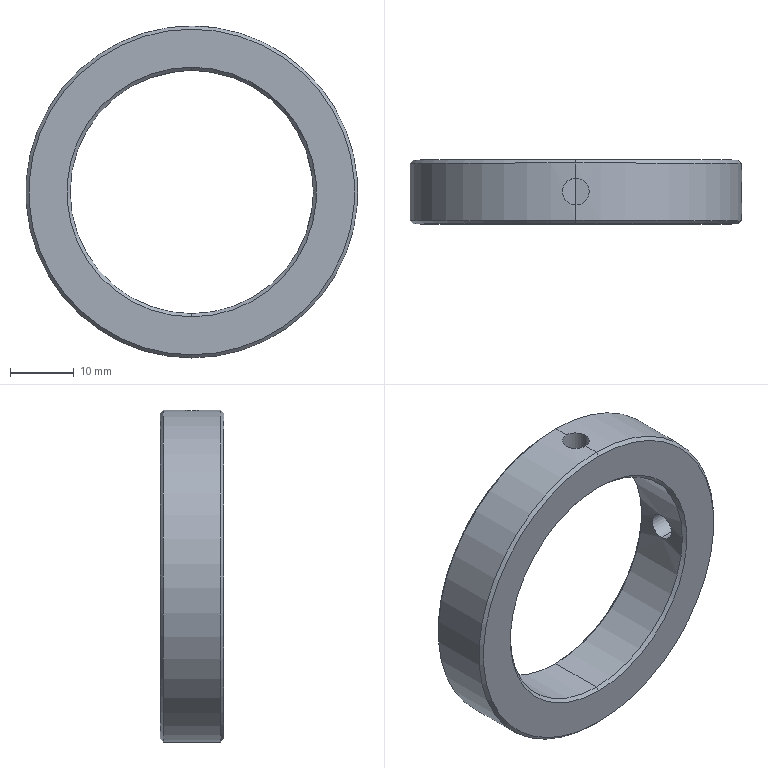Component | SolidWorks | 8TC-A15004-80-19A-1 | 1 solid | 18 faces | box 52 x 10 x 52 mm | volume 9573 mm3 | cylinder 8 | cone 8 | plane 2 | commonest cylinder face diameters 4.2 x4 38.1 x2 52 x2 | material Black Bakelite
build123d program:
from build123d import *

# Parameters (mm, degrees)
SKETCH1_R           = 26
SKETCH1_R_2         = 19.05
BOSS_EXTRUDE1_DEPTH = 5
CHAMFER1_SIZE       = 0.5
SKETCH2_W           = 2.1
SKETCH2_H           = 26
CIRPATTERN1_COUNT   = 2
CIRPATTERN1_ANGLE   = 90


with BuildPart() as part:
    # Sketch1 → Boss-Extrude1 (new, symmetric)
    with BuildSketch(Plane(origin=(0, 0, 0), x_dir=(1, 0, 0), z_dir=(0, 1, 0))):
        with Locations(Location((0, 0, 0), (0, 0, 270))):
            Circle(SKETCH1_R)
        with Locations(Location((0, 0, 0), (0, 0, 270))):
            Circle(SKETCH1_R_2, mode=Mode.SUBTRACT)
    extrude(amount=BOSS_EXTRUDE1_DEPTH, both=True)

    # Chamfer1
    chamfer1_edges = [part.edges().sort_by_distance(p)[0] for p in [
        (0, -5, -26),
        (0, 5, -26),
        (0, -5, -19.05),
        (0, 5, -19.05),
    ]]
    chamfer(chamfer1_edges, length=CHAMFER1_SIZE)

    # Sketch2 → M5 Tapped Hole1 (revolve, cut)
    with BuildSketch(Plane.ZX):
        with Locations((1.05, 13)):
            Rectangle(SKETCH2_W, SKETCH2_H)
    m5_tapped_hole1 = revolve(axis=Axis((-6.35, 0, 0), (1, 0, 0)), mode=Mode.SUBTRACT)

    # CirPattern1: M5 Tapped Hole1 ×2 about axis
    cirpattern1_axis = Axis((0, 5, 0), (0, -1, 0))
    for i in range(1, CIRPATTERN1_COUNT):
        add(m5_tapped_hole1.rotate(cirpattern1_axis, i * CIRPATTERN1_ANGLE / (CIRPATTERN1_COUNT - 1)), mode=Mode.SUBTRACT)


solid = part.part

# Placed as in the assembly
solid = solid.moved(Location((50, 188.5, -500), (0, 0, 0)))
STEP:
#1=CARTESIAN_POINT('',(2.051,7.421,-18.665));
#2=VERTEX_POINT('',#1);
#3=CARTESIAN_POINT('',(1.969,7.339,-18.661));
#4=VERTEX_POINT('',#3);
#5=CARTESIAN_POINT('',(2.051,7.421,-18.665));
#6=CARTESIAN_POINT('',(2.051,7.416,-18.665));
#7=CARTESIAN_POINT('',(2.051,7.41,-18.665));
#8=CARTESIAN_POINT('',(2.049,7.4,-18.665));
#9=CARTESIAN_POINT('',(2.047,7.395,-18.664));
#10=CARTESIAN_POINT('',(2.043,7.385,-18.664));
#11=CARTESIAN_POINT('',(2.04,7.38,-18.664));
#12=CARTESIAN_POINT('',(2.034,7.371,-18.664));
#13=CARTESIAN_POINT('',(2.031,7.367,-18.663));
#14=CARTESIAN_POINT('',(2.023,7.359,-18.663));
#15=CARTESIAN_POINT('',(2.019,7.356,-18.663));
#16=CARTESIAN_POINT('',(2.01,7.35,-18.662));
#17=CARTESIAN_POINT('',(2.005,7.347,-18.662));
#18=CARTESIAN_POINT('',(1.99,7.341,-18.662));
#19=CARTESIAN_POINT('',(1.979,7.339,-18.661));
#20=CARTESIAN_POINT('',(1.969,7.339,-18.661));
#21=B_SPLINE_CURVE_WITH_KNOTS('',3,(#5,#6,#7,#8,#9,#10,#11,#12,#13,#14,#15,#16,#17,#18,#19,#20),.UNSPECIFIED.,.F.,.F.,(4,2,2,2,2,2,2,4),(0.009853,0.01026,0.01067,0.01108,0.01149,0.0119,0.01231,0.01313),.UNSPECIFIED.);
#22=EDGE_CURVE('',#2,#4,#21,.T.);
#23=ORIENTED_EDGE('',*,*,#22,.F.);
#24=CARTESIAN_POINT('',(2.051,7.421,-18.94));
#25=VERTEX_POINT('',#24);
#26=CARTESIAN_POINT('',(2.051,7.421,-19.685));
#27=DIRECTION('',(0.,0.,-1.));
#28=VECTOR('',#27,39.37);
#29=LINE('',#26,#28);
#30=EDGE_CURVE('',#2,#25,#29,.T.);
#31=ORIENTED_EDGE('',*,*,#30,.T.);
#32=CARTESIAN_POINT('',(1.969,7.339,-18.935));
#33=VERTEX_POINT('',#32);
#34=CARTESIAN_POINT('',(2.051,7.421,-18.94));
#35=CARTESIAN_POINT('',(2.051,7.41,-18.94));
#36=CARTESIAN_POINT('',(2.049,7.4,-18.939));
#37=CARTESIAN_POINT('',(2.041,7.38,-18.939));
#38=CARTESIAN_POINT('',(2.035,7.37,-18.938));
#39=CARTESIAN_POINT('',(2.023,7.359,-18.937));
#40=CARTESIAN_POINT('',(2.019,7.356,-18.937));
#41=CARTESIAN_POINT('',(2.01,7.35,-18.936));
#42=CARTESIAN_POINT('',(2.005,7.347,-18.936));
#43=CARTESIAN_POINT('',(1.995,7.343,-18.935));
#44=CARTESIAN_POINT('',(1.99,7.341,-18.935));
#45=CARTESIAN_POINT('',(1.979,7.339,-18.935));
#46=CARTESIAN_POINT('',(1.974,7.339,-18.935));
#47=CARTESIAN_POINT('',(1.969,7.339,-18.935));
#48=B_SPLINE_CURVE_WITH_KNOTS('',3,(#34,#35,#36,#37,#38,#39,#40,#41,#42,#43,#44,#45,#46,#47),.UNSPECIFIED.,.F.,.F.,(4,2,2,2,2,2,4),(0.006571,0.007392,0.008214,0.008624,0.009035,0.009446,0.009857),.UNSPECIFIED.);
#49=EDGE_CURVE('',#25,#33,#48,.T.);
#50=ORIENTED_EDGE('',*,*,#49,.T.);
#51=CARTESIAN_POINT('',(1.886,7.421,-18.94));
#52=VERTEX_POINT('',#51);
#53=CARTESIAN_POINT('',(1.969,7.339,-18.935));
#54=CARTESIAN_POINT('',(1.963,7.339,-18.935));
#55=CARTESIAN_POINT('',(1.958,7.339,-18.935));
#56=CARTESIAN_POINT('',(1.947,7.341,-18.935));
#57=CARTESIAN_POINT('',(1.942,7.343,-18.935));
#58=CARTESIAN_POINT('',(1.932,7.347,-18.936));
#59=CARTESIAN_POINT('',(1.927,7.349,-18.936));
#60=CARTESIAN_POINT('',(1.918,7.355,-18.937));
#61=CARTESIAN_POINT('',(1.914,7.359,-18.937));
#62=CARTESIAN_POINT('',(1.902,7.37,-18.938));
#63=CARTESIAN_POINT('',(1.896,7.38,-18.939));
#64=CARTESIAN_POINT('',(1.888,7.399,-18.939));
#65=CARTESIAN_POINT('',(1.886,7.41,-18.94));
#66=CARTESIAN_POINT('',(1.886,7.421,-18.94));
#67=B_SPLINE_CURVE_WITH_KNOTS('',3,(#53,#54,#55,#56,#57,#58,#59,#60,#61,#62,#63,#64,#65,#66),.UNSPECIFIED.,.F.,.F.,(4,2,2,2,2,2,4),(0.009857,0.01027,0.01068,0.01109,0.0115,0.01232,0.01314),.UNSPECIFIED.);
#68=EDGE_CURVE('',#33,#52,#67,.T.);
#69=ORIENTED_EDGE('',*,*,#68,.T.);
#70=CARTESIAN_POINT('',(1.886,7.421,-18.665));
#71=VERTEX_POINT('',#70);
#72=CARTESIAN_POINT('',(1.886,7.421,-19.685));
#73=DIRECTION('',(0.,0.,-1.));
#74=VECTOR('',#73,39.37);
#75=LINE('',#72,#74);
#76=EDGE_CURVE('',#71,#52,#75,.T.);
#77=ORIENTED_EDGE('',*,*,#76,.F.);
#78=CARTESIAN_POINT('',(1.969,7.339,-18.661));
#79=CARTESIAN_POINT('',(1.963,7.339,-18.661));
#80=CARTESIAN_POINT('',(1.958,7.339,-18.661));
#81=CARTESIAN_POINT('',(1.947,7.341,-18.662));
#82=CARTESIAN_POINT('',(1.942,7.343,-18.662));
#83=CARTESIAN_POINT('',(1.932,7.347,-18.662));
#84=CARTESIAN_POINT('',(1.927,7.35,-18.662));
#85=CARTESIAN_POINT('',(1.918,7.356,-18.663));
#86=CARTESIAN_POINT('',(1.914,7.359,-18.663));
#87=CARTESIAN_POINT('',(1.902,7.37,-18.664));
#88=CARTESIAN_POINT('',(1.896,7.38,-18.664));
#89=CARTESIAN_POINT('',(1.888,7.4,-18.665));
#90=CARTESIAN_POINT('',(1.886,7.41,-18.665));
#91=CARTESIAN_POINT('',(1.886,7.421,-18.665));
#92=B_SPLINE_CURVE_WITH_KNOTS('',3,(#78,#79,#80,#81,#82,#83,#84,#85,#86,#87,#88,#89,#90,#91),.UNSPECIFIED.,.F.,.F.,(4,2,2,2,2,2,4),(0.,0.0004106,0.0008212,0.001232,0.001642,0.002464,0.003285),.UNSPECIFIED.);
#93=EDGE_CURVE('',#4,#71,#92,.T.);
#94=ORIENTED_EDGE('',*,*,#93,.F.);
#95=EDGE_LOOP('',(#23,#31,#50,#69,#77,#94));
#96=FACE_OUTER_BOUND('',#95,.T.);
#97=CARTESIAN_POINT('',(1.969,7.421,-19.685));
#98=DIRECTION('',(0.,0.,-1.));
#99=DIRECTION('',(-1.,0.,0.));
#100=AXIS2_PLACEMENT_3D('',#97,#98,#99);
#101=CYLINDRICAL_SURFACE('',#100,0.08268);
#102=ADVANCED_FACE('',(#96),#101,.F.);
#103=CARTESIAN_POINT('',(2.989,7.421,-19.768));
#104=VERTEX_POINT('',#103);
#105=CARTESIAN_POINT('',(2.989,7.421,-19.602));
#106=VERTEX_POINT('',#105);
#107=CARTESIAN_POINT('',(2.989,7.421,-19.768));
#108=CARTESIAN_POINT('',(2.989,7.416,-19.768));
#109=CARTESIAN_POINT('',(2.989,7.41,-19.767));
#110=CARTESIAN_POINT('',(2.989,7.4,-19.765));
#111=CARTESIAN_POINT('',(2.989,7.395,-19.763));
#112=CARTESIAN_POINT('',(2.989,7.385,-19.759));
#113=CARTESIAN_POINT('',(2.99,7.38,-19.757));
#114=CARTESIAN_POINT('',(2.99,7.371,-19.751));
#115=CARTESIAN_POINT('',(2.99,7.367,-19.747));
#116=CARTESIAN_POINT('',(2.991,7.359,-19.74));
#117=CARTESIAN_POINT('',(2.991,7.356,-19.736));
#118=CARTESIAN_POINT('',(2.991,7.35,-19.726));
#119=CARTESIAN_POINT('',(2.991,7.347,-19.722));
#120=CARTESIAN_POINT('',(2.992,7.341,-19.707));
#121=CARTESIAN_POINT('',(2.992,7.339,-19.696));
#122=CARTESIAN_POINT('',(2.992,7.339,-19.68));
#123=CARTESIAN_POINT('',(2.992,7.339,-19.674));
#124=CARTESIAN_POINT('',(2.992,7.341,-19.664));
#125=CARTESIAN_POINT('',(2.992,7.343,-19.658));
#126=CARTESIAN_POINT('',(2.991,7.347,-19.648));
#127=CARTESIAN_POINT('',(2.991,7.35,-19.644));
#128=CARTESIAN_POINT('',(2.991,7.356,-19.635));
#129=CARTESIAN_POINT('',(2.991,7.359,-19.63));
#130=CARTESIAN_POINT('',(2.99,7.37,-19.619));
#131=CARTESIAN_POINT('',(2.99,7.38,-19.613));
#132=CARTESIAN_POINT('',(2.989,7.4,-19.605));
#133=CARTESIAN_POINT('',(2.989,7.41,-19.602));
#134=CARTESIAN_POINT('',(2.989,7.421,-19.602));
#135=B_SPLINE_CURVE_WITH_KNOTS('',3,(#107,#108,#109,#110,#111,#112,#113,#114,#115,#116,#117,#118,#119,#120,#121,#122,#123,#124,#125,#126,#127,#128,#129,#130,#131,#132,#133,#134),.UNSPECIFIED.,.F.,.F.,(4,2,2,2,2,2,2,2,2,2,2,2,2,4),(0.009853,0.01026,0.01067,0.01108,0.01149,0.01191,0.01232,0.01314,0.01355,0.01396,0.01437,0.01478,0.0156,0.01642),.UNSPECIFIED.);
#136=EDGE_CURVE('',#104,#106,#135,.T.);
#137=ORIENTED_EDGE('',*,*,#136,.F.);
#138=CARTESIAN_POINT('',(2.714,7.421,-19.768));
#139=VERTEX_POINT('',#138);
#140=CARTESIAN_POINT('',(1.969,7.421,-19.768));
#141=DIRECTION('',(-1.,0.,0.));
#142=VECTOR('',#141,39.37);
#143=LINE('',#140,#142);
#144=EDGE_CURVE('',#104,#139,#143,.T.);
#145=ORIENTED_EDGE('',*,*,#144,.T.);
#146=CARTESIAN_POINT('',(2.714,7.421,-19.602));
#147=VERTEX_POINT('',#146);
#148=CARTESIAN_POINT('',(2.714,7.421,-19.768));
#149=CARTESIAN_POINT('',(2.714,7.41,-19.768));
#150=CARTESIAN_POINT('',(2.714,7.4,-19.766));
#151=CARTESIAN_POINT('',(2.715,7.38,-19.757));
#152=CARTESIAN_POINT('',(2.716,7.37,-19.751));
#153=CARTESIAN_POINT('',(2.717,7.359,-19.74));
#154=CARTESIAN_POINT('',(2.717,7.356,-19.735));
#155=CARTESIAN_POINT('',(2.717,7.35,-19.727));
#156=CARTESIAN_POINT('',(2.718,7.347,-19.722));
#157=CARTESIAN_POINT('',(2.718,7.343,-19.712));
#158=CARTESIAN_POINT('',(2.718,7.341,-19.707));
#159=CARTESIAN_POINT('',(2.718,7.339,-19.696));
#160=CARTESIAN_POINT('',(2.719,7.339,-19.691));
#161=CARTESIAN_POINT('',(2.719,7.339,-19.68));
#162=CARTESIAN_POINT('',(2.718,7.339,-19.674));
#163=CARTESIAN_POINT('',(2.718,7.341,-19.664));
#164=CARTESIAN_POINT('',(2.718,7.343,-19.658));
#165=CARTESIAN_POINT('',(2.718,7.347,-19.648));
#166=CARTESIAN_POINT('',(2.717,7.349,-19.644));
#167=CARTESIAN_POINT('',(2.717,7.355,-19.635));
#168=CARTESIAN_POINT('',(2.717,7.359,-19.63));
#169=CARTESIAN_POINT('',(2.716,7.37,-19.619));
#170=CARTESIAN_POINT('',(2.715,7.38,-19.613));
#171=CARTESIAN_POINT('',(2.714,7.399,-19.605));
#172=CARTESIAN_POINT('',(2.714,7.41,-19.602));
#173=CARTESIAN_POINT('',(2.714,7.421,-19.602));
#174=B_SPLINE_CURVE_WITH_KNOTS('',3,(#148,#149,#150,#151,#152,#153,#154,#155,#156,#157,#158,#159,#160,#161,#162,#163,#164,#165,#166,#167,#168,#169,#170,#171,#172,#173),.UNSPECIFIED.,.F.,.F.,(4,2,2,2,2,2,2,2,2,2,2,2,4),(0.006571,0.007392,0.008213,0.008623,0.009034,0.009444,0.009855,0.01027,0.01068,0.01109,0.0115,0.01232,0.01314),.UNSPECIFIED.);
#175=EDGE_CURVE('',#139,#147,#174,.T.);
#176=ORIENTED_EDGE('',*,*,#175,.T.);
#177=CARTESIAN_POINT('',(1.969,7.421,-19.602));
#178=DIRECTION('',(-1.,0.,0.));
#179=VECTOR('',#178,39.37);
#180=LINE('',#177,#179);
#181=EDGE_CURVE('',#106,#147,#180,.T.);
#182=ORIENTED_EDGE('',*,*,#181,.F.);
#183=EDGE_LOOP('',(#137,#145,#176,#182));
#184=FACE_OUTER_BOUND('',#183,.T.);
#185=CARTESIAN_POINT('',(1.969,7.421,-19.685));
#186=DIRECTION('',(-1.,0.,0.));
#187=DIRECTION('',(0.,0.,1.));
#188=AXIS2_PLACEMENT_3D('',#185,#186,#187);
#189=CYLINDRICAL_SURFACE('',#188,0.08268);
#190=ADVANCED_FACE('',(#184),#189,.F.);
#191=CARTESIAN_POINT('',(1.969,7.244,-18.935));
#192=VERTEX_POINT('',#191);
#193=CARTESIAN_POINT('',(1.969,7.244,-20.435));
#194=VERTEX_POINT('',#193);
#195=CARTESIAN_POINT('',(1.969,7.244,-19.685));
#196=DIRECTION('',(0.,-1.,0.));
#197=DIRECTION('',(0.,0.,1.));
#198=AXIS2_PLACEMENT_3D('',#195,#196,#197);
#199=CIRCLE('',#198,0.75);
#200=EDGE_CURVE('',#192,#194,#199,.T.);
#201=ORIENTED_EDGE('',*,*,#200,.F.);
#202=CARTESIAN_POINT('',(1.969,7.224,-18.915));
#203=VERTEX_POINT('',#202);
#204=CARTESIAN_POINT('',(1.969,7.224,-18.915));
#205=DIRECTION('',(0.,-0.7071,0.7071));
#206=VECTOR('',#205,39.37);
#207=LINE('',#204,#206);
#208=EDGE_CURVE('',#192,#203,#207,.T.);
#209=ORIENTED_EDGE('',*,*,#208,.T.);
#210=CARTESIAN_POINT('',(1.969,7.224,-20.455));
#211=VERTEX_POINT('',#210);
#212=CARTESIAN_POINT('',(1.969,7.224,-19.685));
#213=DIRECTION('',(0.,1.,0.));
#214=DIRECTION('',(0.,0.,1.));
#215=AXIS2_PLACEMENT_3D('',#212,#213,#214);
#216=CIRCLE('',#215,0.7697);
#217=EDGE_CURVE('',#211,#203,#216,.T.);
#218=ORIENTED_EDGE('',*,*,#217,.F.);
#219=CARTESIAN_POINT('',(1.969,7.224,-20.455));
#220=DIRECTION('',(0.,-0.7071,-0.7071));
#221=VECTOR('',#220,39.37);
#222=LINE('',#219,#221);
#223=EDGE_CURVE('',#194,#211,#222,.T.);
#224=ORIENTED_EDGE('',*,*,#223,.F.);
#225=EDGE_LOOP('',(#201,#209,#218,#224));
#226=FACE_OUTER_BOUND('',#225,.T.);
#227=CARTESIAN_POINT('',(1.969,7.224,-19.685));
#228=DIRECTION('',(0.,-1.,0.));
#229=DIRECTION('',(0.,0.,-1.));
#230=AXIS2_PLACEMENT_3D('',#227,#228,#229);
#231=CONICAL_SURFACE('',#230,0.7697,0.7854);
#232=ADVANCED_FACE('',(#226),#231,.F.);
#233=CARTESIAN_POINT('',(1.969,7.224,-20.689));
#234=VERTEX_POINT('',#233);
#235=CARTESIAN_POINT('',(1.969,7.224,-18.681));
#236=VERTEX_POINT('',#235);
#237=CARTESIAN_POINT('',(1.969,7.224,-19.685));
#238=DIRECTION('',(0.,-1.,0.));
#239=DIRECTION('',(0.,0.,1.));
#240=AXIS2_PLACEMENT_3D('',#237,#238,#239);
#241=CIRCLE('',#240,1.004);
#242=EDGE_CURVE('',#234,#236,#241,.T.);
#243=ORIENTED_EDGE('',*,*,#242,.F.);
#244=CARTESIAN_POINT('',(1.969,7.244,-20.709));
#245=VERTEX_POINT('',#244);
#246=CARTESIAN_POINT('',(1.969,7.244,-20.709));
#247=DIRECTION('',(0.,0.7071,-0.7071));
#248=VECTOR('',#247,39.37);
#249=LINE('',#246,#248);
#250=EDGE_CURVE('',#234,#245,#249,.T.);
#251=ORIENTED_EDGE('',*,*,#250,.T.);
#252=CARTESIAN_POINT('',(1.969,7.244,-18.661));
#253=VERTEX_POINT('',#252);
#254=CARTESIAN_POINT('',(1.969,7.244,-19.685));
#255=DIRECTION('',(0.,1.,0.));
#256=DIRECTION('',(0.,0.,1.));
#257=AXIS2_PLACEMENT_3D('',#254,#255,#256);
#258=CIRCLE('',#257,1.024);
#259=EDGE_CURVE('',#253,#245,#258,.T.);
#260=ORIENTED_EDGE('',*,*,#259,.F.);
#261=CARTESIAN_POINT('',(1.969,7.244,-18.661));
#262=DIRECTION('',(0.,0.7071,0.7071));
#263=VECTOR('',#262,39.37);
#264=LINE('',#261,#263);
#265=EDGE_CURVE('',#236,#253,#264,.T.);
#266=ORIENTED_EDGE('',*,*,#265,.F.);
#267=EDGE_LOOP('',(#243,#251,#260,#266));
#268=FACE_OUTER_BOUND('',#267,.T.);
#269=CARTESIAN_POINT('',(1.969,7.244,-19.685));
#270=DIRECTION('',(0.,1.,0.));
#271=DIRECTION('',(0.,0.,1.));
#272=AXIS2_PLACEMENT_3D('',#269,#270,#271);
#273=CONICAL_SURFACE('',#272,1.024,0.7854);
#274=ADVANCED_FACE('',(#268),#273,.T.);
#275=CARTESIAN_POINT('',(1.969,7.618,-18.681));
#276=VERTEX_POINT('',#275);
#277=CARTESIAN_POINT('',(1.969,7.618,-20.689));
#278=VERTEX_POINT('',#277);
#279=CARTESIAN_POINT('',(1.969,7.618,-19.685));
#280=DIRECTION('',(0.,1.,0.));
#281=DIRECTION('',(0.,0.,1.));
#282=AXIS2_PLACEMENT_3D('',#279,#280,#281);
#283=CIRCLE('',#282,1.004);
#284=EDGE_CURVE('',#276,#278,#283,.T.);
#285=ORIENTED_EDGE('',*,*,#284,.F.);
#286=CARTESIAN_POINT('',(1.969,7.598,-18.661));
#287=VERTEX_POINT('',#286);
#288=CARTESIAN_POINT('',(1.969,7.618,-18.681));
#289=DIRECTION('',(0.,-0.7071,0.7071));
#290=VECTOR('',#289,39.37);
#291=LINE('',#288,#290);
#292=EDGE_CURVE('',#276,#287,#291,.T.);
#293=ORIENTED_EDGE('',*,*,#292,.T.);
#294=CARTESIAN_POINT('',(1.969,7.598,-20.709));
#295=VERTEX_POINT('',#294);
#296=CARTESIAN_POINT('',(1.969,7.598,-19.685));
#297=DIRECTION('',(0.,-1.,0.));
#298=DIRECTION('',(0.,0.,1.));
#299=AXIS2_PLACEMENT_3D('',#296,#297,#298);
#300=CIRCLE('',#299,1.024);
#301=EDGE_CURVE('',#295,#287,#300,.T.);
#302=ORIENTED_EDGE('',*,*,#301,.F.);
#303=CARTESIAN_POINT('',(1.969,7.618,-20.689));
#304=DIRECTION('',(0.,-0.7071,-0.7071));
#305=VECTOR('',#304,39.37);
#306=LINE('',#303,#305);
#307=EDGE_CURVE('',#278,#295,#306,.T.);
#308=ORIENTED_EDGE('',*,*,#307,.F.);
#309=EDGE_LOOP('',(#285,#293,#302,#308));
#310=FACE_OUTER_BOUND('',#309,.T.);
#311=CARTESIAN_POINT('',(1.969,7.618,-19.685));
#312=DIRECTION('',(0.,-1.,0.));
#313=DIRECTION('',(0.,0.,-1.));
#314=AXIS2_PLACEMENT_3D('',#311,#312,#313);
#315=CONICAL_SURFACE('',#314,1.004,0.7854);
#316=ADVANCED_FACE('',(#310),#315,.T.);
#317=CARTESIAN_POINT('',(1.969,7.598,-20.435));
#318=VERTEX_POINT('',#317);
#319=CARTESIAN_POINT('',(1.969,7.598,-18.935));
#320=VERTEX_POINT('',#319);
#321=CARTESIAN_POINT('',(1.969,7.598,-19.685));
#322=DIRECTION('',(0.,1.,0.));
#323=DIRECTION('',(0.,0.,1.));
#324=AXIS2_PLACEMENT_3D('',#321,#322,#323);
#325=CIRCLE('',#324,0.75);
#326=EDGE_CURVE('',#318,#320,#325,.T.);
#327=ORIENTED_EDGE('',*,*,#326,.F.);
#328=CARTESIAN_POINT('',(1.969,7.618,-20.455));
#329=VERTEX_POINT('',#328);
#330=CARTESIAN_POINT('',(1.969,7.598,-20.435));
#331=DIRECTION('',(0.,0.7071,-0.7071));
#332=VECTOR('',#331,39.37);
#333=LINE('',#330,#332);
#334=EDGE_CURVE('',#318,#329,#333,.T.);
#335=ORIENTED_EDGE('',*,*,#334,.T.);
#336=CARTESIAN_POINT('',(1.969,7.618,-18.915));
#337=VERTEX_POINT('',#336);
#338=CARTESIAN_POINT('',(1.969,7.618,-19.685));
#339=DIRECTION('',(0.,-1.,0.));
#340=DIRECTION('',(0.,0.,1.));
#341=AXIS2_PLACEMENT_3D('',#338,#339,#340);
#342=CIRCLE('',#341,0.7697);
#343=EDGE_CURVE('',#337,#329,#342,.T.);
#344=ORIENTED_EDGE('',*,*,#343,.F.);
#345=CARTESIAN_POINT('',(1.969,7.598,-18.935));
#346=DIRECTION('',(0.,0.7071,0.7071));
#347=VECTOR('',#346,39.37);
#348=LINE('',#345,#347);
#349=EDGE_CURVE('',#320,#337,#348,.T.);
#350=ORIENTED_EDGE('',*,*,#349,.F.);
#351=EDGE_LOOP('',(#327,#335,#344,#350));
#352=FACE_OUTER_BOUND('',#351,.T.);
#353=CARTESIAN_POINT('',(1.969,7.598,-19.685));
#354=DIRECTION('',(0.,1.,0.));
#355=DIRECTION('',(0.,0.,1.));
#356=AXIS2_PLACEMENT_3D('',#353,#354,#355);
#357=CONICAL_SURFACE('',#356,0.75,0.7854);
#358=ADVANCED_FACE('',(#352),#357,.F.);
#359=ORIENTED_EDGE('',*,*,#326,.T.);
#360=CARTESIAN_POINT('',(1.969,7.504,-18.935));
#361=VERTEX_POINT('',#360);
#362=CARTESIAN_POINT('',(1.969,7.618,-18.935));
#363=DIRECTION('',(0.,-1.,0.));
#364=VECTOR('',#363,39.37);
#365=LINE('',#362,#364);
#366=EDGE_CURVE('',#320,#361,#365,.T.);
#367=ORIENTED_EDGE('',*,*,#366,.T.);
#368=CARTESIAN_POINT('',(1.886,7.421,-18.94));
#369=CARTESIAN_POINT('',(1.886,7.427,-18.94));
#370=CARTESIAN_POINT('',(1.886,7.432,-18.94));
#371=CARTESIAN_POINT('',(1.888,7.443,-18.939));
#372=CARTESIAN_POINT('',(1.89,7.448,-18.939));
#373=CARTESIAN_POINT('',(1.894,7.458,-18.939));
#374=CARTESIAN_POINT('',(1.897,7.463,-18.938));
#375=CARTESIAN_POINT('',(1.903,7.472,-18.938));
#376=CARTESIAN_POINT('',(1.906,7.476,-18.938));
#377=CARTESIAN_POINT('',(1.918,7.487,-18.937));
#378=CARTESIAN_POINT('',(1.927,7.494,-18.936));
#379=CARTESIAN_POINT('',(1.947,7.502,-18.935));
#380=CARTESIAN_POINT('',(1.958,7.504,-18.935));
#381=CARTESIAN_POINT('',(1.969,7.504,-18.935));
#382=B_SPLINE_CURVE_WITH_KNOTS('',3,(#368,#369,#370,#371,#372,#373,#374,#375,#376,#377,#378,#379,#380,#381),.UNSPECIFIED.,.F.,.F.,(4,2,2,2,2,2,4),(0.,0.0004108,0.0008215,0.001232,0.001643,0.002465,0.003286),.UNSPECIFIED.);
#383=EDGE_CURVE('',#52,#361,#382,.T.);
#384=ORIENTED_EDGE('',*,*,#383,.F.);
#385=ORIENTED_EDGE('',*,*,#68,.F.);
#386=CARTESIAN_POINT('',(1.969,7.618,-18.935));
#387=DIRECTION('',(0.,-1.,0.));
#388=VECTOR('',#387,39.37);
#389=LINE('',#386,#388);
#390=EDGE_CURVE('',#33,#192,#389,.T.);
#391=ORIENTED_EDGE('',*,*,#390,.T.);
#392=ORIENTED_EDGE('',*,*,#200,.T.);
#393=CARTESIAN_POINT('',(1.969,7.618,-20.435));
#394=DIRECTION('',(0.,-1.,0.));
#395=VECTOR('',#394,39.37);
#396=LINE('',#393,#395);
#397=EDGE_CURVE('',#318,#194,#396,.T.);
#398=ORIENTED_EDGE('',*,*,#397,.F.);
#399=EDGE_LOOP('',(#359,#367,#384,#385,#391,#392,#398));
#400=FACE_OUTER_BOUND('',#399,.T.);
#401=CARTESIAN_POINT('',(1.969,7.618,-19.685));
#402=DIRECTION('',(0.,-1.,0.));
#403=DIRECTION('',(0.,0.,-1.));
#404=AXIS2_PLACEMENT_3D('',#401,#402,#403);
#405=CYLINDRICAL_SURFACE('',#404,0.75);
#406=ADVANCED_FACE('',(#400),#405,.F.);
#407=CARTESIAN_POINT('',(2.989,7.421,-19.602));
#408=CARTESIAN_POINT('',(2.989,7.427,-19.602));
#409=CARTESIAN_POINT('',(2.989,7.432,-19.603));
#410=CARTESIAN_POINT('',(2.989,7.443,-19.605));
#411=CARTESIAN_POINT('',(2.989,7.448,-19.607));
#412=CARTESIAN_POINT('',(2.989,7.458,-19.611));
#413=CARTESIAN_POINT('',(2.99,7.463,-19.613));
#414=CARTESIAN_POINT('',(2.99,7.472,-19.619));
#415=CARTESIAN_POINT('',(2.99,7.476,-19.623));
#416=CARTESIAN_POINT('',(2.991,7.484,-19.63));
#417=CARTESIAN_POINT('',(2.991,7.487,-19.635));
#418=CARTESIAN_POINT('',(2.991,7.493,-19.644));
#419=CARTESIAN_POINT('',(2.991,7.496,-19.648));
#420=CARTESIAN_POINT('',(2.992,7.5,-19.658));
#421=CARTESIAN_POINT('',(2.992,7.501,-19.664));
#422=CARTESIAN_POINT('',(2.992,7.503,-19.674));
#423=CARTESIAN_POINT('',(2.992,7.504,-19.68));
#424=CARTESIAN_POINT('',(2.992,7.504,-19.696));
#425=CARTESIAN_POINT('',(2.992,7.502,-19.707));
#426=CARTESIAN_POINT('',(2.991,7.494,-19.727));
#427=CARTESIAN_POINT('',(2.991,7.487,-19.736));
#428=CARTESIAN_POINT('',(2.99,7.476,-19.747));
#429=CARTESIAN_POINT('',(2.99,7.472,-19.751));
#430=CARTESIAN_POINT('',(2.99,7.463,-19.757));
#431=CARTESIAN_POINT('',(2.989,7.458,-19.759));
#432=CARTESIAN_POINT('',(2.989,7.448,-19.763));
#433=CARTESIAN_POINT('',(2.989,7.443,-19.765));
#434=CARTESIAN_POINT('',(2.989,7.432,-19.767));
#435=CARTESIAN_POINT('',(2.989,7.427,-19.768));
#436=CARTESIAN_POINT('',(2.989,7.421,-19.768));
#437=B_SPLINE_CURVE_WITH_KNOTS('',3,(#407,#408,#409,#410,#411,#412,#413,#414,#415,#416,#417,#418,#419,#420,#421,#422,#423,#424,#425,#426,#427,#428,#429,#430,#431,#432,#433,#434,#435,#436),.UNSPECIFIED.,.F.,.F.,(4,2,2,2,2,2,2,2,2,2,2,2,2,2,4),(0.003285,0.003695,0.004106,0.004516,0.004927,0.005337,0.005748,0.006159,0.006569,0.00739,0.008211,0.008622,0.009032,0.009443,0.009853),.UNSPECIFIED.);
#438=EDGE_CURVE('',#106,#104,#437,.T.);
#439=ORIENTED_EDGE('',*,*,#438,.T.);
#440=ORIENTED_EDGE('',*,*,#136,.T.);
#441=EDGE_LOOP('',(#439,#440));
#442=FACE_BOUND('',#441,.T.);
#443=ORIENTED_EDGE('',*,*,#301,.T.);
#444=CARTESIAN_POINT('',(1.969,7.504,-18.661));
#445=VERTEX_POINT('',#444);
#446=CARTESIAN_POINT('',(1.969,7.618,-18.661));
#447=DIRECTION('',(0.,-1.,0.));
#448=VECTOR('',#447,39.37);
#449=LINE('',#446,#448);
#450=EDGE_CURVE('',#287,#445,#449,.T.);
#451=ORIENTED_EDGE('',*,*,#450,.T.);
#452=CARTESIAN_POINT('',(1.969,7.504,-18.661));
#453=CARTESIAN_POINT('',(1.979,7.504,-18.661));
#454=CARTESIAN_POINT('',(1.99,7.502,-18.662));
#455=CARTESIAN_POINT('',(2.01,7.494,-18.662));
#456=CARTESIAN_POINT('',(2.019,7.487,-18.663));
#457=CARTESIAN_POINT('',(2.031,7.476,-18.663));
#458=CARTESIAN_POINT('',(2.034,7.472,-18.664));
#459=CARTESIAN_POINT('',(2.04,7.463,-18.664));
#460=CARTESIAN_POINT('',(2.043,7.458,-18.664));
#461=CARTESIAN_POINT('',(2.047,7.448,-18.664));
#462=CARTESIAN_POINT('',(2.049,7.443,-18.665));
#463=CARTESIAN_POINT('',(2.051,7.432,-18.665));
#464=CARTESIAN_POINT('',(2.051,7.427,-18.665));
#465=CARTESIAN_POINT('',(2.051,7.421,-18.665));
#466=B_SPLINE_CURVE_WITH_KNOTS('',3,(#452,#453,#454,#455,#456,#457,#458,#459,#460,#461,#462,#463,#464,#465),.UNSPECIFIED.,.F.,.F.,(4,2,2,2,2,2,4),(0.006568,0.007389,0.008211,0.008621,0.009032,0.009443,0.009853),.UNSPECIFIED.);
#467=EDGE_CURVE('',#445,#2,#466,.T.);
#468=ORIENTED_EDGE('',*,*,#467,.T.);
#469=ORIENTED_EDGE('',*,*,#22,.T.);
#470=CARTESIAN_POINT('',(1.969,7.618,-18.661));
#471=DIRECTION('',(0.,-1.,0.));
#472=VECTOR('',#471,39.37);
#473=LINE('',#470,#472);
#474=EDGE_CURVE('',#4,#253,#473,.T.);
#475=ORIENTED_EDGE('',*,*,#474,.T.);
#476=ORIENTED_EDGE('',*,*,#259,.T.);
#477=CARTESIAN_POINT('',(1.969,7.618,-20.709));
#478=DIRECTION('',(0.,-1.,0.));
#479=VECTOR('',#478,39.37);
#480=LINE('',#477,#479);
#481=EDGE_CURVE('',#295,#245,#480,.T.);
#482=ORIENTED_EDGE('',*,*,#481,.F.);
#483=EDGE_LOOP('',(#443,#451,#468,#469,#475,#476,#482));
#484=FACE_OUTER_BOUND('',#483,.T.);
#485=CARTESIAN_POINT('',(1.969,7.618,-19.685));
#486=DIRECTION('',(0.,-1.,0.));
#487=DIRECTION('',(0.,0.,-1.));
#488=AXIS2_PLACEMENT_3D('',#485,#486,#487);
#489=CYLINDRICAL_SURFACE('',#488,1.024);
#490=ADVANCED_FACE('',(#442,#484),#489,.T.);
#491=ORIENTED_EDGE('',*,*,#343,.T.);
#492=CARTESIAN_POINT('',(1.969,7.618,-19.685));
#493=DIRECTION('',(0.,-1.,0.));
#494=DIRECTION('',(0.,0.,1.));
#495=AXIS2_PLACEMENT_3D('',#492,#493,#494);
#496=CIRCLE('',#495,0.7697);
#497=EDGE_CURVE('',#329,#337,#496,.T.);
#498=ORIENTED_EDGE('',*,*,#497,.T.);
#499=EDGE_LOOP('',(#491,#498));
#500=FACE_BOUND('',#499,.T.);
#501=CARTESIAN_POINT('',(1.969,7.618,-19.685));
#502=DIRECTION('',(0.,1.,0.));
#503=DIRECTION('',(0.,0.,1.));
#504=AXIS2_PLACEMENT_3D('',#501,#502,#503);
#505=CIRCLE('',#504,1.004);
#506=EDGE_CURVE('',#278,#276,#505,.T.);
#507=ORIENTED_EDGE('',*,*,#506,.T.);
#508=ORIENTED_EDGE('',*,*,#284,.T.);
#509=EDGE_LOOP('',(#507,#508));
#510=FACE_OUTER_BOUND('',#509,.T.);
#511=CARTESIAN_POINT('',(1.969,7.618,-19.685));
#512=DIRECTION('',(0.,1.,0.));
#513=DIRECTION('',(0.,0.,1.));
#514=AXIS2_PLACEMENT_3D('',#511,#512,#513);
#515=PLANE('',#514);
#516=ADVANCED_FACE('',(#500,#510),#515,.T.);
#517=CARTESIAN_POINT('',(1.969,7.224,-19.685));
#518=DIRECTION('',(0.,-1.,0.));
#519=DIRECTION('',(0.,0.,1.));
#520=AXIS2_PLACEMENT_3D('',#517,#518,#519);
#521=CIRCLE('',#520,1.004);
#522=EDGE_CURVE('',#236,#234,#521,.T.);
#523=ORIENTED_EDGE('',*,*,#522,.T.);
#524=ORIENTED_EDGE('',*,*,#242,.T.);
#525=EDGE_LOOP('',(#523,#524));
#526=FACE_OUTER_BOUND('',#525,.T.);
#527=ORIENTED_EDGE('',*,*,#217,.T.);
#528=CARTESIAN_POINT('',(1.969,7.224,-19.685));
#529=DIRECTION('',(0.,1.,0.));
#530=DIRECTION('',(0.,0.,1.));
#531=AXIS2_PLACEMENT_3D('',#528,#529,#530);
#532=CIRCLE('',#531,0.7697);
#533=EDGE_CURVE('',#203,#211,#532,.T.);
#534=ORIENTED_EDGE('',*,*,#533,.T.);
#535=EDGE_LOOP('',(#527,#534));
#536=FACE_BOUND('',#535,.T.);
#537=CARTESIAN_POINT('',(1.969,7.224,-19.685));
#538=DIRECTION('',(0.,1.,0.));
#539=DIRECTION('',(0.,0.,1.));
#540=AXIS2_PLACEMENT_3D('',#537,#538,#539);
#541=PLANE('',#540);
#542=ADVANCED_FACE('',(#526,#536),#541,.F.);
#543=ORIENTED_EDGE('',*,*,#450,.F.);
#544=CARTESIAN_POINT('',(1.969,7.598,-19.685));
#545=DIRECTION('',(0.,-1.,0.));
#546=DIRECTION('',(0.,0.,1.));
#547=AXIS2_PLACEMENT_3D('',#544,#545,#546);
#548=CIRCLE('',#547,1.024);
#549=EDGE_CURVE('',#287,#295,#548,.T.);
#550=ORIENTED_EDGE('',*,*,#549,.T.);
#551=ORIENTED_EDGE('',*,*,#481,.T.);
#552=CARTESIAN_POINT('',(1.969,7.244,-19.685));
#553=DIRECTION('',(0.,1.,0.));
#554=DIRECTION('',(0.,0.,1.));
#555=AXIS2_PLACEMENT_3D('',#552,#553,#554);
#556=CIRCLE('',#555,1.024);
#557=EDGE_CURVE('',#245,#253,#556,.T.);
#558=ORIENTED_EDGE('',*,*,#557,.T.);
#559=ORIENTED_EDGE('',*,*,#474,.F.);
#560=ORIENTED_EDGE('',*,*,#93,.T.);
#561=CARTESIAN_POINT('',(1.886,7.421,-18.665));
#562=CARTESIAN_POINT('',(1.886,7.427,-18.665));
#563=CARTESIAN_POINT('',(1.886,7.432,-18.665));
#564=CARTESIAN_POINT('',(1.888,7.443,-18.665));
#565=CARTESIAN_POINT('',(1.89,7.448,-18.664));
#566=CARTESIAN_POINT('',(1.894,7.458,-18.664));
#567=CARTESIAN_POINT('',(1.897,7.463,-18.664));
#568=CARTESIAN_POINT('',(1.903,7.472,-18.664));
#569=CARTESIAN_POINT('',(1.906,7.476,-18.663));
#570=CARTESIAN_POINT('',(1.914,7.484,-18.663));
#571=CARTESIAN_POINT('',(1.918,7.487,-18.663));
#572=CARTESIAN_POINT('',(1.927,7.493,-18.662));
#573=CARTESIAN_POINT('',(1.932,7.496,-18.662));
#574=CARTESIAN_POINT('',(1.942,7.5,-18.662));
#575=CARTESIAN_POINT('',(1.947,7.501,-18.662));
#576=CARTESIAN_POINT('',(1.958,7.503,-18.661));
#577=CARTESIAN_POINT('',(1.963,7.504,-18.661));
#578=CARTESIAN_POINT('',(1.969,7.504,-18.661));
#579=B_SPLINE_CURVE_WITH_KNOTS('',3,(#561,#562,#563,#564,#565,#566,#567,#568,#569,#570,#571,#572,#573,#574,#575,#576,#577,#578),.UNSPECIFIED.,.F.,.F.,(4,2,2,2,2,2,2,2,4),(0.003285,0.003695,0.004106,0.004516,0.004927,0.005337,0.005747,0.006158,0.006568),.UNSPECIFIED.);
#580=EDGE_CURVE('',#71,#445,#579,.T.);
#581=ORIENTED_EDGE('',*,*,#580,.T.);
#582=EDGE_LOOP('',(#543,#550,#551,#558,#559,#560,#581));
#583=FACE_OUTER_BOUND('',#582,.T.);
#584=CARTESIAN_POINT('',(1.969,7.618,-19.685));
#585=DIRECTION('',(0.,-1.,0.));
#586=DIRECTION('',(0.,0.,-1.));
#587=AXIS2_PLACEMENT_3D('',#584,#585,#586);
#588=CYLINDRICAL_SURFACE('',#587,1.024);
#589=ADVANCED_FACE('',(#583),#588,.T.);
#590=ORIENTED_EDGE('',*,*,#366,.F.);
#591=CARTESIAN_POINT('',(1.969,7.598,-19.685));
#592=DIRECTION('',(0.,1.,0.));
#593=DIRECTION('',(0.,0.,1.));
#594=AXIS2_PLACEMENT_3D('',#591,#592,#593);
#595=CIRCLE('',#594,0.75);
#596=EDGE_CURVE('',#320,#318,#595,.T.);
#597=ORIENTED_EDGE('',*,*,#596,.T.);
#598=ORIENTED_EDGE('',*,*,#397,.T.);
#599=CARTESIAN_POINT('',(1.969,7.244,-19.685));
#600=DIRECTION('',(0.,-1.,0.));
#601=DIRECTION('',(0.,0.,1.));
#602=AXIS2_PLACEMENT_3D('',#599,#600,#601);
#603=CIRCLE('',#602,0.75);
#604=EDGE_CURVE('',#194,#192,#603,.T.);
#605=ORIENTED_EDGE('',*,*,#604,.T.);
#606=ORIENTED_EDGE('',*,*,#390,.F.);
#607=ORIENTED_EDGE('',*,*,#49,.F.);
#608=CARTESIAN_POINT('',(1.969,7.504,-18.935));
#609=CARTESIAN_POINT('',(1.974,7.504,-18.935));
#610=CARTESIAN_POINT('',(1.979,7.503,-18.935));
#611=CARTESIAN_POINT('',(1.99,7.501,-18.935));
#612=CARTESIAN_POINT('',(1.995,7.5,-18.935));
#613=CARTESIAN_POINT('',(2.005,7.496,-18.936));
#614=CARTESIAN_POINT('',(2.01,7.493,-18.936));
#615=CARTESIAN_POINT('',(2.019,7.487,-18.937));
#616=CARTESIAN_POINT('',(2.023,7.484,-18.937));
#617=CARTESIAN_POINT('',(2.031,7.476,-18.938));
#618=CARTESIAN_POINT('',(2.034,7.472,-18.938));
#619=CARTESIAN_POINT('',(2.04,7.463,-18.938));
#620=CARTESIAN_POINT('',(2.043,7.458,-18.939));
#621=CARTESIAN_POINT('',(2.047,7.448,-18.939));
#622=CARTESIAN_POINT('',(2.049,7.443,-18.939));
#623=CARTESIAN_POINT('',(2.051,7.432,-18.94));
#624=CARTESIAN_POINT('',(2.051,7.427,-18.94));
#625=CARTESIAN_POINT('',(2.051,7.421,-18.94));
#626=B_SPLINE_CURVE_WITH_KNOTS('',3,(#608,#609,#610,#611,#612,#613,#614,#615,#616,#617,#618,#619,#620,#621,#622,#623,#624,#625),.UNSPECIFIED.,.F.,.F.,(4,2,2,2,2,2,2,2,4),(0.003286,0.003697,0.004107,0.004518,0.004928,0.005339,0.005749,0.00616,0.006571),.UNSPECIFIED.);
#627=EDGE_CURVE('',#361,#25,#626,.T.);
#628=ORIENTED_EDGE('',*,*,#627,.F.);
#629=EDGE_LOOP('',(#590,#597,#598,#605,#606,#607,#628));
#630=FACE_OUTER_BOUND('',#629,.T.);
#631=CARTESIAN_POINT('',(2.714,7.421,-19.602));
#632=CARTESIAN_POINT('',(2.714,7.427,-19.602));
#633=CARTESIAN_POINT('',(2.714,7.432,-19.603));
#634=CARTESIAN_POINT('',(2.714,7.443,-19.605));
#635=CARTESIAN_POINT('',(2.714,7.448,-19.607));
#636=CARTESIAN_POINT('',(2.715,7.458,-19.611));
#637=CARTESIAN_POINT('',(2.715,7.463,-19.613));
#638=CARTESIAN_POINT('',(2.716,7.472,-19.619));
#639=CARTESIAN_POINT('',(2.716,7.476,-19.623));
#640=CARTESIAN_POINT('',(2.717,7.487,-19.634));
#641=CARTESIAN_POINT('',(2.717,7.494,-19.643));
#642=CARTESIAN_POINT('',(2.718,7.502,-19.663));
#643=CARTESIAN_POINT('',(2.719,7.504,-19.674));
#644=CARTESIAN_POINT('',(2.719,7.504,-19.69));
#645=CARTESIAN_POINT('',(2.718,7.503,-19.696));
#646=CARTESIAN_POINT('',(2.718,7.501,-19.706));
#647=CARTESIAN_POINT('',(2.718,7.5,-19.712));
#648=CARTESIAN_POINT('',(2.718,7.496,-19.722));
#649=CARTESIAN_POINT('',(2.717,7.493,-19.727));
#650=CARTESIAN_POINT('',(2.717,7.487,-19.735));
#651=CARTESIAN_POINT('',(2.717,7.484,-19.74));
#652=CARTESIAN_POINT('',(2.716,7.476,-19.747));
#653=CARTESIAN_POINT('',(2.716,7.472,-19.751));
#654=CARTESIAN_POINT('',(2.715,7.463,-19.757));
#655=CARTESIAN_POINT('',(2.715,7.458,-19.759));
#656=CARTESIAN_POINT('',(2.714,7.448,-19.763));
#657=CARTESIAN_POINT('',(2.714,7.443,-19.765));
#658=CARTESIAN_POINT('',(2.714,7.432,-19.767));
#659=CARTESIAN_POINT('',(2.714,7.427,-19.768));
#660=CARTESIAN_POINT('',(2.714,7.421,-19.768));
#661=B_SPLINE_CURVE_WITH_KNOTS('',3,(#631,#632,#633,#634,#635,#636,#637,#638,#639,#640,#641,#642,#643,#644,#645,#646,#647,#648,#649,#650,#651,#652,#653,#654,#655,#656,#657,#658,#659,#660),.UNSPECIFIED.,.F.,.F.,(4,2,2,2,2,2,2,2,2,2,2,2,2,2,4),(0.,0.0004107,0.0008213,0.001232,0.001643,0.002464,0.003285,0.003696,0.004107,0.004517,0.004928,0.005339,0.005749,0.00616,0.006571),.UNSPECIFIED.);
#662=EDGE_CURVE('',#147,#139,#661,.T.);
#663=ORIENTED_EDGE('',*,*,#662,.F.);
#664=ORIENTED_EDGE('',*,*,#175,.F.);
#665=EDGE_LOOP('',(#663,#664));
#666=FACE_BOUND('',#665,.T.);
#667=CARTESIAN_POINT('',(1.969,7.618,-19.685));
#668=DIRECTION('',(0.,-1.,0.));
#669=DIRECTION('',(0.,0.,-1.));
#670=AXIS2_PLACEMENT_3D('',#667,#668,#669);
#671=CYLINDRICAL_SURFACE('',#670,0.75);
#672=ADVANCED_FACE('',(#630,#666),#671,.F.);
#673=ORIENTED_EDGE('',*,*,#334,.F.);
#674=ORIENTED_EDGE('',*,*,#596,.F.);
#675=ORIENTED_EDGE('',*,*,#349,.T.);
#676=ORIENTED_EDGE('',*,*,#497,.F.);
#677=EDGE_LOOP('',(#673,#674,#675,#676));
#678=FACE_OUTER_BOUND('',#677,.T.);
#679=CARTESIAN_POINT('',(1.969,7.598,-19.685));
#680=DIRECTION('',(0.,1.,0.));
#681=DIRECTION('',(0.,0.,1.));
#682=AXIS2_PLACEMENT_3D('',#679,#680,#681);
#683=CONICAL_SURFACE('',#682,0.75,0.7854);
#684=ADVANCED_FACE('',(#678),#683,.F.);
#685=ORIENTED_EDGE('',*,*,#292,.F.);
#686=ORIENTED_EDGE('',*,*,#506,.F.);
#687=ORIENTED_EDGE('',*,*,#307,.T.);
#688=ORIENTED_EDGE('',*,*,#549,.F.);
#689=EDGE_LOOP('',(#685,#686,#687,#688));
#690=FACE_OUTER_BOUND('',#689,.T.);
#691=CARTESIAN_POINT('',(1.969,7.618,-19.685));
#692=DIRECTION('',(0.,-1.,0.));
#693=DIRECTION('',(0.,0.,-1.));
#694=AXIS2_PLACEMENT_3D('',#691,#692,#693);
#695=CONICAL_SURFACE('',#694,1.004,0.7854);
#696=ADVANCED_FACE('',(#690),#695,.T.);
#697=ORIENTED_EDGE('',*,*,#250,.F.);
#698=ORIENTED_EDGE('',*,*,#522,.F.);
#699=ORIENTED_EDGE('',*,*,#265,.T.);
#700=ORIENTED_EDGE('',*,*,#557,.F.);
#701=EDGE_LOOP('',(#697,#698,#699,#700));
#702=FACE_OUTER_BOUND('',#701,.T.);
#703=CARTESIAN_POINT('',(1.969,7.244,-19.685));
#704=DIRECTION('',(0.,1.,0.));
#705=DIRECTION('',(0.,0.,1.));
#706=AXIS2_PLACEMENT_3D('',#703,#704,#705);
#707=CONICAL_SURFACE('',#706,1.024,0.7854);
#708=ADVANCED_FACE('',(#702),#707,.T.);
#709=ORIENTED_EDGE('',*,*,#208,.F.);
#710=ORIENTED_EDGE('',*,*,#604,.F.);
#711=ORIENTED_EDGE('',*,*,#223,.T.);
#712=ORIENTED_EDGE('',*,*,#533,.F.);
#713=EDGE_LOOP('',(#709,#710,#711,#712));
#714=FACE_OUTER_BOUND('',#713,.T.);
#715=CARTESIAN_POINT('',(1.969,7.224,-19.685));
#716=DIRECTION('',(0.,-1.,0.));
#717=DIRECTION('',(0.,0.,-1.));
#718=AXIS2_PLACEMENT_3D('',#715,#716,#717);
#719=CONICAL_SURFACE('',#718,0.7697,0.7854);
#720=ADVANCED_FACE('',(#714),#719,.F.);
#721=ORIENTED_EDGE('',*,*,#144,.F.);
#722=ORIENTED_EDGE('',*,*,#438,.F.);
#723=ORIENTED_EDGE('',*,*,#181,.T.);
#724=ORIENTED_EDGE('',*,*,#662,.T.);
#725=EDGE_LOOP('',(#721,#722,#723,#724));
#726=FACE_OUTER_BOUND('',#725,.T.);
#727=CARTESIAN_POINT('',(1.969,7.421,-19.685));
#728=DIRECTION('',(-1.,0.,0.));
#729=DIRECTION('',(0.,0.,1.));
#730=AXIS2_PLACEMENT_3D('',#727,#728,#729);
#731=CYLINDRICAL_SURFACE('',#730,0.08268);
#732=ADVANCED_FACE('',(#726),#731,.F.);
#733=ORIENTED_EDGE('',*,*,#30,.F.);
#734=ORIENTED_EDGE('',*,*,#467,.F.);
#735=ORIENTED_EDGE('',*,*,#580,.F.);
#736=ORIENTED_EDGE('',*,*,#76,.T.);
#737=ORIENTED_EDGE('',*,*,#383,.T.);
#738=ORIENTED_EDGE('',*,*,#627,.T.);
#739=EDGE_LOOP('',(#733,#734,#735,#736,#737,#738));
#740=FACE_OUTER_BOUND('',#739,.T.);
#741=CARTESIAN_POINT('',(1.969,7.421,-19.685));
#742=DIRECTION('',(0.,0.,-1.));
#743=DIRECTION('',(-1.,0.,0.));
#744=AXIS2_PLACEMENT_3D('',#741,#742,#743);
#745=CYLINDRICAL_SURFACE('',#744,0.08268);
#746=ADVANCED_FACE('',(#740),#745,.F.);
#747=CLOSED_SHELL('',(#102,#190,#232,#274,#316,#358,#406,#490,#516,#542,#589,#672,#684,#696,#708,#720,#732,#746));
#748=MANIFOLD_SOLID_BREP('',#747);
#749=CARTESIAN_POINT('',(0.,0.,0.));
#750=DIRECTION('',(0.,0.,1.));
#751=DIRECTION('',(1.,0.,0.));
#752=AXIS2_PLACEMENT_3D('',#749,#750,#751);
#753=(LENGTH_UNIT()NAMED_UNIT(*)SI_UNIT($,.METRE.));
#754=LENGTH_MEASURE_WITH_UNIT(LENGTH_MEASURE(0.0254),#753);
#755=DIMENSIONAL_EXPONENTS(1.,0.,0.,0.,0.,0.,0.);
#756=(CONVERSION_BASED_UNIT('',#754)LENGTH_UNIT()NAMED_UNIT(#755));
#757=UNCERTAINTY_MEASURE_WITH_UNIT(LENGTH_MEASURE(0.00001),#756,'','');
#758=(NAMED_UNIT(*)PLANE_ANGLE_UNIT()SI_UNIT($,.RADIAN.));
#759=(NAMED_UNIT(*)SI_UNIT($,.STERADIAN.)SOLID_ANGLE_UNIT());
#760=(GEOMETRIC_REPRESENTATION_CONTEXT(3)GLOBAL_UNCERTAINTY_ASSIGNED_CONTEXT((#757))GLOBAL_UNIT_ASSIGNED_CONTEXT((#756,#758,#759))REPRESENTATION_CONTEXT('',''));
#761=ADVANCED_BREP_SHAPE_REPRESENTATION('',(#748,#752),#760);
#762=COLOUR_RGB('',0.7922,0.8196,0.9333);
#763=FILL_AREA_STYLE_COLOUR('',#762);
#764=FILL_AREA_STYLE('',(#763));
#765=SURFACE_STYLE_FILL_AREA(#764);
#766=SURFACE_SIDE_STYLE('',(#765));
#767=SURFACE_STYLE_USAGE(.BOTH.,#766);
#768=PRESENTATION_STYLE_ASSIGNMENT((#767));
#769=STYLED_ITEM('',(#768),#748);
#770=PRESENTATION_LAYER_ASSIGNMENT('','',(#769));
#771=(LENGTH_UNIT()NAMED_UNIT(*)SI_UNIT($,.METRE.));
#772=LENGTH_MEASURE_WITH_UNIT(LENGTH_MEASURE(0.0254),#771);
#773=DIMENSIONAL_EXPONENTS(1.,0.,0.,0.,0.,0.,0.);
#774=(CONVERSION_BASED_UNIT('',#772)LENGTH_UNIT()NAMED_UNIT(#773));
#775=UNCERTAINTY_MEASURE_WITH_UNIT(LENGTH_MEASURE(0.00001),#774,'','');
#776=(NAMED_UNIT(*)PLANE_ANGLE_UNIT()SI_UNIT($,.RADIAN.));
#777=(NAMED_UNIT(*)SI_UNIT($,.STERADIAN.)SOLID_ANGLE_UNIT());
#778=(GEOMETRIC_REPRESENTATION_CONTEXT(3)GLOBAL_UNCERTAINTY_ASSIGNED_CONTEXT((#775))GLOBAL_UNIT_ASSIGNED_CONTEXT((#774,#776,#777))REPRESENTATION_CONTEXT('',''));
#779=MECHANICAL_DESIGN_GEOMETRIC_PRESENTATION_REPRESENTATION('',(#769),#778);